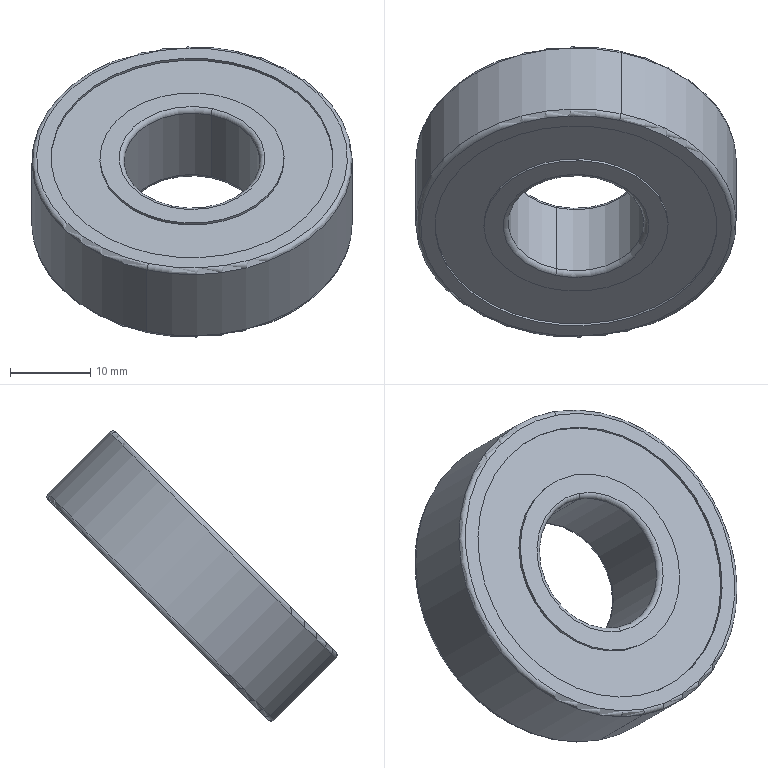Component | SolidWorks | AssemblyDriveAxis-1_6203-2 | 1 solid | 26 faces | box 40 x 36.27 x 36.27 mm | volume 11947 mm3 | cylinder 12 | torus 8 | plane 6 | commonest cylinder face diameters 35.2 x4 23 x4 40 x2 17 x2
build123d program:
from build123d import *


with BuildPart() as part:
    # Sketch1 → Revolve1 (revolve)
    with BuildSketch(Plane.XY, mode=Mode.PRIVATE) as revolve1_sk:
        with BuildLine():
            Line((0, 19.4), (0, 17.6))
            Line((0, 17.6), (0.342, 17.6))
            Line((0.342, 17.6), (0.342, 11.5))
            Line((0.342, 11.5), (0, 11.5))
            Line((0, 11.5), (0, 9.1))
            ThreePointArc((0, 9.1), (0.1757, 8.676), (0.6, 8.5))
            Line((0.6, 8.5), (11.4, 8.5))
            ThreePointArc((11.4, 8.5), (11.824, 8.676), (12, 9.1))
            Line((12, 9.1), (12, 11.5))
            Line((12, 11.5), (11.658, 11.5))
            Line((11.658, 11.5), (11.658, 17.6))
            Line((11.658, 17.6), (12, 17.6))
            Line((12, 17.6), (12, 19.4))
            ThreePointArc((12, 19.4), (11.824, 19.824), (11.4, 20))
            Line((11.4, 20), (0.6, 20))
            ThreePointArc((0.6, 20), (0.1757, 19.824), (0, 19.4))
        make_face()
    revolve(revolve1_sk.sketch.rotate(Axis((12, 0, 0), (-1, 0, 0)), 270), axis=Axis((12, 0, 0), (-1, 0, 0)))


solid = part.part

# Placed as in the assembly
solid = solid.moved(Location((-102, 782.057, 125.043), (135, 86.529, 90)))
STEP:
#1=COLOUR_RGB('',0.7922,0.8196,0.9333);
#2=FILL_AREA_STYLE_COLOUR('',#1);
#3=FILL_AREA_STYLE('',(#2));
#4=SURFACE_STYLE_FILL_AREA(#3);
#5=SURFACE_SIDE_STYLE('',(#4));
#6=SURFACE_STYLE_USAGE(.BOTH.,#5);
#7=PRESENTATION_STYLE_ASSIGNMENT((#6));
#8=CARTESIAN_POINT('',(-4.237,30.239,4.405));
#9=VERTEX_POINT('',#8);
#10=CARTESIAN_POINT('',(-3.794,31.307,5.474));
#11=VERTEX_POINT('',#10);
#12=CARTESIAN_POINT('',(-4.016,30.773,4.94));
#13=DIRECTION('',(-0.,-0.7071,0.7071));
#14=DIRECTION('',(-0.2811,-0.6786,-0.6786));
#15=AXIS2_PLACEMENT_3D('',#12,#13,#14);
#16=CIRCLE('',#15,0.7874);
#17=EDGE_CURVE('',#9,#11,#16,.T.);
#18=ORIENTED_EDGE('',*,*,#17,.T.);
#19=CARTESIAN_POINT('',(-3.794,31.007,5.775));
#20=VERTEX_POINT('',#19);
#21=CARTESIAN_POINT('',(-3.794,31.324,5.457));
#22=DIRECTION('',(-0.,-0.7071,0.7071));
#23=VECTOR('',#22,39.37);
#24=LINE('',#21,#23);
#25=EDGE_CURVE('',#11,#20,#24,.T.);
#26=ORIENTED_EDGE('',*,*,#25,.T.);
#27=CARTESIAN_POINT('',(-4.237,29.938,4.706));
#28=VERTEX_POINT('',#27);
#29=CARTESIAN_POINT('',(-4.016,30.472,5.24));
#30=DIRECTION('',(-0.,-0.7071,0.7071));
#31=DIRECTION('',(-0.2811,-0.6786,-0.6786));
#32=AXIS2_PLACEMENT_3D('',#29,#30,#31);
#33=CIRCLE('',#32,0.7874);
#34=EDGE_CURVE('',#28,#20,#33,.T.);
#35=ORIENTED_EDGE('',*,*,#34,.F.);
#36=CARTESIAN_POINT('',(-4.237,30.255,4.389));
#37=DIRECTION('',(-0.,-0.7071,0.7071));
#38=VECTOR('',#37,39.37);
#39=LINE('',#36,#38);
#40=EDGE_CURVE('',#9,#28,#39,.T.);
#41=ORIENTED_EDGE('',*,*,#40,.F.);
#42=EDGE_LOOP('',(#18,#26,#35,#41));
#43=FACE_OUTER_BOUND('',#42,.T.);
#44=CARTESIAN_POINT('',(-4.016,30.79,4.923));
#45=DIRECTION('',(-0.,-0.7071,0.7071));
#46=DIRECTION('',(-0.2811,-0.6786,-0.6786));
#47=AXIS2_PLACEMENT_3D('',#44,#45,#46);
#48=CYLINDRICAL_SURFACE('',#47,0.7874);
#49=ADVANCED_FACE('',(#43),#48,.T.);
#50=CARTESIAN_POINT('',(-4.23,30.271,4.405));
#51=VERTEX_POINT('',#50);
#52=CARTESIAN_POINT('',(-3.801,31.308,5.441));
#53=VERTEX_POINT('',#52);
#54=CARTESIAN_POINT('',(-4.016,30.79,4.923));
#55=DIRECTION('',(-0.,-0.7071,0.7071));
#56=DIRECTION('',(-0.2811,-0.6786,-0.6786));
#57=AXIS2_PLACEMENT_3D('',#54,#55,#56);
#58=CIRCLE('',#57,0.7638);
#59=EDGE_CURVE('',#51,#53,#58,.T.);
#60=ORIENTED_EDGE('',*,*,#59,.T.);
#61=CARTESIAN_POINT('',(-3.801,31.291,5.458));
#62=DIRECTION('',(0.9597,-0.1988,-0.1988));
#63=DIRECTION('',(-0.2028,0.,-0.9792));
#64=AXIS2_PLACEMENT_3D('',#61,#62,#63);
#65=CIRCLE('',#64,0.02362);
#66=EDGE_CURVE('',#53,#11,#65,.T.);
#67=ORIENTED_EDGE('',*,*,#66,.T.);
#68=ORIENTED_EDGE('',*,*,#17,.F.);
#69=CARTESIAN_POINT('',(-4.23,30.255,4.421));
#70=DIRECTION('',(-0.9597,0.1988,0.1988));
#71=DIRECTION('',(0.2028,0.,0.9792));
#72=AXIS2_PLACEMENT_3D('',#69,#70,#71);
#73=CIRCLE('',#72,0.02362);
#74=EDGE_CURVE('',#51,#9,#73,.T.);
#75=ORIENTED_EDGE('',*,*,#74,.F.);
#76=EDGE_LOOP('',(#60,#67,#68,#75));
#77=FACE_OUTER_BOUND('',#76,.T.);
#78=CARTESIAN_POINT('',(-4.016,30.773,4.94));
#79=DIRECTION('',(-0.,-0.7071,0.7071));
#80=DIRECTION('',(-0.2811,-0.6786,-0.6786));
#81=AXIS2_PLACEMENT_3D('',#78,#79,#80);
#82=TOROIDAL_SURFACE('',#81,0.7638,0.02362);
#83=ADVANCED_FACE('',(#77),#82,.T.);
#84=CARTESIAN_POINT('',(-3.821,31.26,5.393));
#85=VERTEX_POINT('',#84);
#86=CARTESIAN_POINT('',(-4.211,30.319,4.453));
#87=VERTEX_POINT('',#86);
#88=CARTESIAN_POINT('',(-4.016,30.79,4.923));
#89=DIRECTION('',(-0.,-0.7071,0.7071));
#90=DIRECTION('',(-0.2811,-0.6786,-0.6786));
#91=AXIS2_PLACEMENT_3D('',#88,#89,#90);
#92=CIRCLE('',#91,0.6929);
#93=EDGE_CURVE('',#85,#87,#92,.T.);
#94=ORIENTED_EDGE('',*,*,#93,.F.);
#95=CARTESIAN_POINT('',(-3.821,31.25,5.403));
#96=VERTEX_POINT('',#95);
#97=CARTESIAN_POINT('',(-3.821,31.26,5.393));
#98=DIRECTION('',(-0.,-0.7071,0.7071));
#99=VECTOR('',#98,39.37);
#100=LINE('',#97,#99);
#101=EDGE_CURVE('',#85,#96,#100,.T.);
#102=ORIENTED_EDGE('',*,*,#101,.T.);
#103=CARTESIAN_POINT('',(-4.211,30.31,4.462));
#104=VERTEX_POINT('',#103);
#105=CARTESIAN_POINT('',(-4.016,30.78,4.932));
#106=DIRECTION('',(-0.,-0.7071,0.7071));
#107=DIRECTION('',(-0.2811,-0.6786,-0.6786));
#108=AXIS2_PLACEMENT_3D('',#105,#106,#107);
#109=CIRCLE('',#108,0.6929);
#110=EDGE_CURVE('',#96,#104,#109,.T.);
#111=ORIENTED_EDGE('',*,*,#110,.T.);
#112=CARTESIAN_POINT('',(-4.211,30.319,4.453));
#113=DIRECTION('',(-0.,-0.7071,0.7071));
#114=VECTOR('',#113,39.37);
#115=LINE('',#112,#114);
#116=EDGE_CURVE('',#87,#104,#115,.T.);
#117=ORIENTED_EDGE('',*,*,#116,.F.);
#118=EDGE_LOOP('',(#94,#102,#111,#117));
#119=FACE_OUTER_BOUND('',#118,.T.);
#120=CARTESIAN_POINT('',(-4.016,30.79,4.923));
#121=DIRECTION('',(-0.,-0.7071,0.7071));
#122=DIRECTION('',(-0.2811,-0.6786,-0.6786));
#123=AXIS2_PLACEMENT_3D('',#120,#121,#122);
#124=CYLINDRICAL_SURFACE('',#123,0.6929);
#125=ADVANCED_FACE('',(#119),#124,.F.);
#126=CARTESIAN_POINT('',(-4.143,30.482,4.616));
#127=VERTEX_POINT('',#126);
#128=CARTESIAN_POINT('',(-3.888,31.097,5.23));
#129=VERTEX_POINT('',#128);
#130=CARTESIAN_POINT('',(-4.016,30.79,4.923));
#131=DIRECTION('',(-0.,-0.7071,0.7071));
#132=DIRECTION('',(-0.2811,-0.6786,-0.6786));
#133=AXIS2_PLACEMENT_3D('',#130,#131,#132);
#134=CIRCLE('',#133,0.4528);
#135=EDGE_CURVE('',#127,#129,#134,.T.);
#136=ORIENTED_EDGE('',*,*,#135,.T.);
#137=CARTESIAN_POINT('',(-3.888,31.087,5.24));
#138=VERTEX_POINT('',#137);
#139=CARTESIAN_POINT('',(-3.888,31.097,5.23));
#140=DIRECTION('',(-0.,-0.7071,0.7071));
#141=VECTOR('',#140,39.37);
#142=LINE('',#139,#141);
#143=EDGE_CURVE('',#129,#138,#142,.T.);
#144=ORIENTED_EDGE('',*,*,#143,.T.);
#145=CARTESIAN_POINT('',(-4.143,30.473,4.625));
#146=VERTEX_POINT('',#145);
#147=CARTESIAN_POINT('',(-4.016,30.78,4.932));
#148=DIRECTION('',(-0.,-0.7071,0.7071));
#149=DIRECTION('',(-0.2811,-0.6786,-0.6786));
#150=AXIS2_PLACEMENT_3D('',#147,#148,#149);
#151=CIRCLE('',#150,0.4528);
#152=EDGE_CURVE('',#146,#138,#151,.T.);
#153=ORIENTED_EDGE('',*,*,#152,.F.);
#154=CARTESIAN_POINT('',(-4.143,30.482,4.616));
#155=DIRECTION('',(-0.,-0.7071,0.7071));
#156=VECTOR('',#155,39.37);
#157=LINE('',#154,#156);
#158=EDGE_CURVE('',#127,#146,#157,.T.);
#159=ORIENTED_EDGE('',*,*,#158,.F.);
#160=EDGE_LOOP('',(#136,#144,#153,#159));
#161=FACE_OUTER_BOUND('',#160,.T.);
#162=CARTESIAN_POINT('',(-4.016,30.79,4.923));
#163=DIRECTION('',(-0.,-0.7071,0.7071));
#164=DIRECTION('',(-0.2811,-0.6786,-0.6786));
#165=AXIS2_PLACEMENT_3D('',#162,#163,#164);
#166=CYLINDRICAL_SURFACE('',#165,0.4528);
#167=ADVANCED_FACE('',(#161),#166,.T.);
#168=CARTESIAN_POINT('',(-4.11,30.546,4.713));
#169=VERTEX_POINT('',#168);
#170=CARTESIAN_POINT('',(-3.922,31.,5.167));
#171=VERTEX_POINT('',#170);
#172=CARTESIAN_POINT('',(-4.016,30.773,4.94));
#173=DIRECTION('',(-0.,-0.7071,0.7071));
#174=DIRECTION('',(-0.2811,-0.6786,-0.6786));
#175=AXIS2_PLACEMENT_3D('',#172,#173,#174);
#176=CIRCLE('',#175,0.3346);
#177=EDGE_CURVE('',#169,#171,#176,.T.);
#178=ORIENTED_EDGE('',*,*,#177,.T.);
#179=CARTESIAN_POINT('',(-3.915,31.033,5.166));
#180=VERTEX_POINT('',#179);
#181=CARTESIAN_POINT('',(-3.915,31.016,5.183));
#182=DIRECTION('',(0.9597,-0.1988,-0.1988));
#183=DIRECTION('',(-0.2028,0.,-0.9792));
#184=AXIS2_PLACEMENT_3D('',#181,#182,#183);
#185=CIRCLE('',#184,0.02362);
#186=EDGE_CURVE('',#171,#180,#185,.T.);
#187=ORIENTED_EDGE('',*,*,#186,.T.);
#188=CARTESIAN_POINT('',(-4.116,30.547,4.68));
#189=VERTEX_POINT('',#188);
#190=CARTESIAN_POINT('',(-4.016,30.79,4.923));
#191=DIRECTION('',(-0.,-0.7071,0.7071));
#192=DIRECTION('',(-0.2811,-0.6786,-0.6786));
#193=AXIS2_PLACEMENT_3D('',#190,#191,#192);
#194=CIRCLE('',#193,0.3583);
#195=EDGE_CURVE('',#189,#180,#194,.T.);
#196=ORIENTED_EDGE('',*,*,#195,.F.);
#197=CARTESIAN_POINT('',(-4.116,30.53,4.697));
#198=DIRECTION('',(-0.9597,0.1988,0.1988));
#199=DIRECTION('',(0.2028,0.,0.9792));
#200=AXIS2_PLACEMENT_3D('',#197,#198,#199);
#201=CIRCLE('',#200,0.02362);
#202=EDGE_CURVE('',#169,#189,#201,.T.);
#203=ORIENTED_EDGE('',*,*,#202,.F.);
#204=EDGE_LOOP('',(#178,#187,#196,#203));
#205=FACE_OUTER_BOUND('',#204,.T.);
#206=CARTESIAN_POINT('',(-4.016,30.773,4.94));
#207=DIRECTION('',(-0.,-0.7071,0.7071));
#208=DIRECTION('',(-0.2811,-0.6786,-0.6786));
#209=AXIS2_PLACEMENT_3D('',#206,#207,#208);
#210=TOROIDAL_SURFACE('',#209,0.3583,0.02362);
#211=ADVANCED_FACE('',(#205),#210,.T.);
#212=CARTESIAN_POINT('',(-4.016,30.773,4.94));
#213=DIRECTION('',(-0.,-0.7071,0.7071));
#214=DIRECTION('',(-0.2811,-0.6786,-0.6786));
#215=AXIS2_PLACEMENT_3D('',#212,#213,#214);
#216=CIRCLE('',#215,0.3346);
#217=EDGE_CURVE('',#171,#169,#216,.T.);
#218=ORIENTED_EDGE('',*,*,#217,.F.);
#219=CARTESIAN_POINT('',(-3.922,30.699,5.467));
#220=VERTEX_POINT('',#219);
#221=CARTESIAN_POINT('',(-3.922,31.017,5.15));
#222=DIRECTION('',(-0.,-0.7071,0.7071));
#223=VECTOR('',#222,39.37);
#224=LINE('',#221,#223);
#225=EDGE_CURVE('',#171,#220,#224,.T.);
#226=ORIENTED_EDGE('',*,*,#225,.T.);
#227=CARTESIAN_POINT('',(-4.11,30.245,5.013));
#228=VERTEX_POINT('',#227);
#229=CARTESIAN_POINT('',(-4.016,30.472,5.24));
#230=DIRECTION('',(-0.,-0.7071,0.7071));
#231=DIRECTION('',(-0.2811,-0.6786,-0.6786));
#232=AXIS2_PLACEMENT_3D('',#229,#230,#231);
#233=CIRCLE('',#232,0.3346);
#234=EDGE_CURVE('',#220,#228,#233,.T.);
#235=ORIENTED_EDGE('',*,*,#234,.T.);
#236=CARTESIAN_POINT('',(-4.11,30.563,4.696));
#237=DIRECTION('',(-0.,-0.7071,0.7071));
#238=VECTOR('',#237,39.37);
#239=LINE('',#236,#238);
#240=EDGE_CURVE('',#169,#228,#239,.T.);
#241=ORIENTED_EDGE('',*,*,#240,.F.);
#242=EDGE_LOOP('',(#218,#226,#235,#241));
#243=FACE_OUTER_BOUND('',#242,.T.);
#244=CARTESIAN_POINT('',(-4.016,30.79,4.923));
#245=DIRECTION('',(-0.,-0.7071,0.7071));
#246=DIRECTION('',(-0.2811,-0.6786,-0.6786));
#247=AXIS2_PLACEMENT_3D('',#244,#245,#246);
#248=CYLINDRICAL_SURFACE('',#247,0.3346);
#249=ADVANCED_FACE('',(#243),#248,.F.);
#250=CARTESIAN_POINT('',(-4.116,30.212,5.014));
#251=VERTEX_POINT('',#250);
#252=CARTESIAN_POINT('',(-3.915,30.699,5.5));
#253=VERTEX_POINT('',#252);
#254=CARTESIAN_POINT('',(-4.016,30.456,5.257));
#255=DIRECTION('',(-0.,-0.7071,0.7071));
#256=DIRECTION('',(-0.2811,-0.6786,-0.6786));
#257=AXIS2_PLACEMENT_3D('',#254,#255,#256);
#258=CIRCLE('',#257,0.3583);
#259=EDGE_CURVE('',#251,#253,#258,.T.);
#260=ORIENTED_EDGE('',*,*,#259,.T.);
#261=CARTESIAN_POINT('',(-3.915,30.715,5.483));
#262=DIRECTION('',(0.9597,-0.1988,-0.1988));
#263=DIRECTION('',(-0.2028,0.,-0.9792));
#264=AXIS2_PLACEMENT_3D('',#261,#262,#263);
#265=CIRCLE('',#264,0.02362);
#266=EDGE_CURVE('',#253,#220,#265,.T.);
#267=ORIENTED_EDGE('',*,*,#266,.T.);
#268=CARTESIAN_POINT('',(-4.016,30.472,5.24));
#269=DIRECTION('',(-0.,-0.7071,0.7071));
#270=DIRECTION('',(-0.2811,-0.6786,-0.6786));
#271=AXIS2_PLACEMENT_3D('',#268,#269,#270);
#272=CIRCLE('',#271,0.3346);
#273=EDGE_CURVE('',#228,#220,#272,.T.);
#274=ORIENTED_EDGE('',*,*,#273,.F.);
#275=CARTESIAN_POINT('',(-4.116,30.229,4.997));
#276=DIRECTION('',(-0.9597,0.1988,0.1988));
#277=DIRECTION('',(0.2028,0.,0.9792));
#278=AXIS2_PLACEMENT_3D('',#275,#276,#277);
#279=CIRCLE('',#278,0.02362);
#280=EDGE_CURVE('',#251,#228,#279,.T.);
#281=ORIENTED_EDGE('',*,*,#280,.F.);
#282=EDGE_LOOP('',(#260,#267,#274,#281));
#283=FACE_OUTER_BOUND('',#282,.T.);
#284=CARTESIAN_POINT('',(-4.016,30.472,5.24));
#285=DIRECTION('',(-0.,-0.7071,0.7071));
#286=DIRECTION('',(-0.2811,-0.6786,-0.6786));
#287=AXIS2_PLACEMENT_3D('',#284,#285,#286);
#288=TOROIDAL_SURFACE('',#287,0.3583,0.02362);
#289=ADVANCED_FACE('',(#283),#288,.T.);
#290=CARTESIAN_POINT('',(-4.143,30.158,4.94));
#291=VERTEX_POINT('',#290);
#292=CARTESIAN_POINT('',(-3.888,30.772,5.555));
#293=VERTEX_POINT('',#292);
#294=CARTESIAN_POINT('',(-4.016,30.465,5.247));
#295=DIRECTION('',(-0.,-0.7071,0.7071));
#296=DIRECTION('',(-0.2811,-0.6786,-0.6786));
#297=AXIS2_PLACEMENT_3D('',#294,#295,#296);
#298=CIRCLE('',#297,0.4528);
#299=EDGE_CURVE('',#291,#293,#298,.T.);
#300=ORIENTED_EDGE('',*,*,#299,.T.);
#301=CARTESIAN_POINT('',(-3.888,30.763,5.564));
#302=VERTEX_POINT('',#301);
#303=CARTESIAN_POINT('',(-3.888,31.097,5.23));
#304=DIRECTION('',(-0.,-0.7071,0.7071));
#305=VECTOR('',#304,39.37);
#306=LINE('',#303,#305);
#307=EDGE_CURVE('',#293,#302,#306,.T.);
#308=ORIENTED_EDGE('',*,*,#307,.T.);
#309=CARTESIAN_POINT('',(-4.143,30.148,4.95));
#310=VERTEX_POINT('',#309);
#311=CARTESIAN_POINT('',(-4.016,30.456,5.257));
#312=DIRECTION('',(-0.,-0.7071,0.7071));
#313=DIRECTION('',(-0.2811,-0.6786,-0.6786));
#314=AXIS2_PLACEMENT_3D('',#311,#312,#313);
#315=CIRCLE('',#314,0.4528);
#316=EDGE_CURVE('',#310,#302,#315,.T.);
#317=ORIENTED_EDGE('',*,*,#316,.F.);
#318=CARTESIAN_POINT('',(-4.143,30.482,4.616));
#319=DIRECTION('',(-0.,-0.7071,0.7071));
#320=VECTOR('',#319,39.37);
#321=LINE('',#318,#320);
#322=EDGE_CURVE('',#291,#310,#321,.T.);
#323=ORIENTED_EDGE('',*,*,#322,.F.);
#324=EDGE_LOOP('',(#300,#308,#317,#323));
#325=FACE_OUTER_BOUND('',#324,.T.);
#326=CARTESIAN_POINT('',(-4.016,30.79,4.923));
#327=DIRECTION('',(-0.,-0.7071,0.7071));
#328=DIRECTION('',(-0.2811,-0.6786,-0.6786));
#329=AXIS2_PLACEMENT_3D('',#326,#327,#328);
#330=CYLINDRICAL_SURFACE('',#329,0.4528);
#331=ADVANCED_FACE('',(#325),#330,.T.);
#332=CARTESIAN_POINT('',(-3.821,30.935,5.718));
#333=VERTEX_POINT('',#332);
#334=CARTESIAN_POINT('',(-4.211,29.995,4.777));
#335=VERTEX_POINT('',#334);
#336=CARTESIAN_POINT('',(-4.016,30.465,5.247));
#337=DIRECTION('',(-0.,-0.7071,0.7071));
#338=DIRECTION('',(-0.2811,-0.6786,-0.6786));
#339=AXIS2_PLACEMENT_3D('',#336,#337,#338);
#340=CIRCLE('',#339,0.6929);
#341=EDGE_CURVE('',#333,#335,#340,.T.);
#342=ORIENTED_EDGE('',*,*,#341,.F.);
#343=CARTESIAN_POINT('',(-3.821,30.926,5.727));
#344=VERTEX_POINT('',#343);
#345=CARTESIAN_POINT('',(-3.821,31.26,5.393));
#346=DIRECTION('',(-0.,-0.7071,0.7071));
#347=VECTOR('',#346,39.37);
#348=LINE('',#345,#347);
#349=EDGE_CURVE('',#333,#344,#348,.T.);
#350=ORIENTED_EDGE('',*,*,#349,.T.);
#351=CARTESIAN_POINT('',(-4.211,29.985,4.787));
#352=VERTEX_POINT('',#351);
#353=CARTESIAN_POINT('',(-4.016,30.456,5.257));
#354=DIRECTION('',(-0.,-0.7071,0.7071));
#355=DIRECTION('',(-0.2811,-0.6786,-0.6786));
#356=AXIS2_PLACEMENT_3D('',#353,#354,#355);
#357=CIRCLE('',#356,0.6929);
#358=EDGE_CURVE('',#344,#352,#357,.T.);
#359=ORIENTED_EDGE('',*,*,#358,.T.);
#360=CARTESIAN_POINT('',(-4.211,30.319,4.453));
#361=DIRECTION('',(-0.,-0.7071,0.7071));
#362=VECTOR('',#361,39.37);
#363=LINE('',#360,#362);
#364=EDGE_CURVE('',#335,#352,#363,.T.);
#365=ORIENTED_EDGE('',*,*,#364,.F.);
#366=EDGE_LOOP('',(#342,#350,#359,#365));
#367=FACE_OUTER_BOUND('',#366,.T.);
#368=CARTESIAN_POINT('',(-4.016,30.79,4.923));
#369=DIRECTION('',(-0.,-0.7071,0.7071));
#370=DIRECTION('',(-0.2811,-0.6786,-0.6786));
#371=AXIS2_PLACEMENT_3D('',#368,#369,#370);
#372=CYLINDRICAL_SURFACE('',#371,0.6929);
#373=ADVANCED_FACE('',(#367),#372,.F.);
#374=ORIENTED_EDGE('',*,*,#34,.T.);
#375=CARTESIAN_POINT('',(-3.801,30.974,5.775));
#376=VERTEX_POINT('',#375);
#377=CARTESIAN_POINT('',(-3.801,30.991,5.759));
#378=DIRECTION('',(0.9597,-0.1988,-0.1988));
#379=DIRECTION('',(-0.2028,0.,-0.9792));
#380=AXIS2_PLACEMENT_3D('',#377,#378,#379);
#381=CIRCLE('',#380,0.02362);
#382=EDGE_CURVE('',#20,#376,#381,.T.);
#383=ORIENTED_EDGE('',*,*,#382,.T.);
#384=CARTESIAN_POINT('',(-4.23,29.937,4.739));
#385=VERTEX_POINT('',#384);
#386=CARTESIAN_POINT('',(-4.016,30.456,5.257));
#387=DIRECTION('',(-0.,-0.7071,0.7071));
#388=DIRECTION('',(-0.2811,-0.6786,-0.6786));
#389=AXIS2_PLACEMENT_3D('',#386,#387,#388);
#390=CIRCLE('',#389,0.7638);
#391=EDGE_CURVE('',#385,#376,#390,.T.);
#392=ORIENTED_EDGE('',*,*,#391,.F.);
#393=CARTESIAN_POINT('',(-4.23,29.954,4.722));
#394=DIRECTION('',(-0.9597,0.1988,0.1988));
#395=DIRECTION('',(0.2028,0.,0.9792));
#396=AXIS2_PLACEMENT_3D('',#393,#394,#395);
#397=CIRCLE('',#396,0.02362);
#398=EDGE_CURVE('',#28,#385,#397,.T.);
#399=ORIENTED_EDGE('',*,*,#398,.F.);
#400=EDGE_LOOP('',(#374,#383,#392,#399));
#401=FACE_OUTER_BOUND('',#400,.T.);
#402=CARTESIAN_POINT('',(-4.016,30.472,5.24));
#403=DIRECTION('',(-0.,-0.7071,0.7071));
#404=DIRECTION('',(-0.2811,-0.6786,-0.6786));
#405=AXIS2_PLACEMENT_3D('',#402,#403,#404);
#406=TOROIDAL_SURFACE('',#405,0.7638,0.02362);
#407=ADVANCED_FACE('',(#401),#406,.T.);
#408=ORIENTED_EDGE('',*,*,#382,.F.);
#409=CARTESIAN_POINT('',(-4.016,30.472,5.24));
#410=DIRECTION('',(-0.,-0.7071,0.7071));
#411=DIRECTION('',(-0.2811,-0.6786,-0.6786));
#412=AXIS2_PLACEMENT_3D('',#409,#410,#411);
#413=CIRCLE('',#412,0.7874);
#414=EDGE_CURVE('',#20,#28,#413,.T.);
#415=ORIENTED_EDGE('',*,*,#414,.T.);
#416=ORIENTED_EDGE('',*,*,#398,.T.);
#417=CARTESIAN_POINT('',(-4.016,30.456,5.257));
#418=DIRECTION('',(-0.,-0.7071,0.7071));
#419=DIRECTION('',(-0.2811,-0.6786,-0.6786));
#420=AXIS2_PLACEMENT_3D('',#417,#418,#419);
#421=CIRCLE('',#420,0.7638);
#422=EDGE_CURVE('',#376,#385,#421,.T.);
#423=ORIENTED_EDGE('',*,*,#422,.F.);
#424=EDGE_LOOP('',(#408,#415,#416,#423));
#425=FACE_OUTER_BOUND('',#424,.T.);
#426=CARTESIAN_POINT('',(-4.016,30.472,5.24));
#427=DIRECTION('',(-0.,-0.7071,0.7071));
#428=DIRECTION('',(-0.2811,-0.6786,-0.6786));
#429=AXIS2_PLACEMENT_3D('',#426,#427,#428);
#430=TOROIDAL_SURFACE('',#429,0.7638,0.02362);
#431=ADVANCED_FACE('',(#425),#430,.T.);
#432=CARTESIAN_POINT('',(-4.016,30.456,5.257));
#433=DIRECTION('',(-0.,-0.7071,0.7071));
#434=DIRECTION('',(-0.2811,-0.6786,-0.6786));
#435=AXIS2_PLACEMENT_3D('',#432,#433,#434);
#436=CIRCLE('',#435,0.6929);
#437=EDGE_CURVE('',#352,#344,#436,.T.);
#438=ORIENTED_EDGE('',*,*,#437,.F.);
#439=ORIENTED_EDGE('',*,*,#358,.F.);
#440=EDGE_LOOP('',(#438,#439));
#441=FACE_BOUND('',#440,.T.);
#442=ORIENTED_EDGE('',*,*,#391,.T.);
#443=ORIENTED_EDGE('',*,*,#422,.T.);
#444=EDGE_LOOP('',(#442,#443));
#445=FACE_OUTER_BOUND('',#444,.T.);
#446=CARTESIAN_POINT('',(-3.283,30.304,5.105));
#447=DIRECTION('',(0.,0.7071,-0.7071));
#448=DIRECTION('',(0.2811,0.6786,0.6786));
#449=AXIS2_PLACEMENT_3D('',#446,#447,#448);
#450=PLANE('',#449);
#451=ADVANCED_FACE('',(#441,#445),#450,.F.);
#452=ORIENTED_EDGE('',*,*,#349,.F.);
#453=CARTESIAN_POINT('',(-4.016,30.465,5.247));
#454=DIRECTION('',(-0.,-0.7071,0.7071));
#455=DIRECTION('',(-0.2811,-0.6786,-0.6786));
#456=AXIS2_PLACEMENT_3D('',#453,#454,#455);
#457=CIRCLE('',#456,0.6929);
#458=EDGE_CURVE('',#335,#333,#457,.T.);
#459=ORIENTED_EDGE('',*,*,#458,.F.);
#460=ORIENTED_EDGE('',*,*,#364,.T.);
#461=ORIENTED_EDGE('',*,*,#437,.T.);
#462=EDGE_LOOP('',(#452,#459,#460,#461));
#463=FACE_OUTER_BOUND('',#462,.T.);
#464=CARTESIAN_POINT('',(-4.016,30.79,4.923));
#465=DIRECTION('',(-0.,-0.7071,0.7071));
#466=DIRECTION('',(-0.2811,-0.6786,-0.6786));
#467=AXIS2_PLACEMENT_3D('',#464,#465,#466);
#468=CYLINDRICAL_SURFACE('',#467,0.6929);
#469=ADVANCED_FACE('',(#463),#468,.F.);
#470=ORIENTED_EDGE('',*,*,#299,.F.);
#471=CARTESIAN_POINT('',(-4.016,30.465,5.247));
#472=DIRECTION('',(-0.,-0.7071,0.7071));
#473=DIRECTION('',(-0.2811,-0.6786,-0.6786));
#474=AXIS2_PLACEMENT_3D('',#471,#472,#473);
#475=CIRCLE('',#474,0.4528);
#476=EDGE_CURVE('',#293,#291,#475,.T.);
#477=ORIENTED_EDGE('',*,*,#476,.F.);
#478=EDGE_LOOP('',(#470,#477));
#479=FACE_BOUND('',#478,.T.);
#480=ORIENTED_EDGE('',*,*,#458,.T.);
#481=ORIENTED_EDGE('',*,*,#341,.T.);
#482=EDGE_LOOP('',(#480,#481));
#483=FACE_OUTER_BOUND('',#482,.T.);
#484=CARTESIAN_POINT('',(-3.351,30.327,5.11));
#485=DIRECTION('',(0.,0.7071,-0.7071));
#486=DIRECTION('',(0.2811,0.6786,0.6786));
#487=AXIS2_PLACEMENT_3D('',#484,#485,#486);
#488=PLANE('',#487);
#489=ADVANCED_FACE('',(#479,#483),#488,.F.);
#490=ORIENTED_EDGE('',*,*,#307,.F.);
#491=ORIENTED_EDGE('',*,*,#476,.T.);
#492=ORIENTED_EDGE('',*,*,#322,.T.);
#493=CARTESIAN_POINT('',(-4.016,30.456,5.257));
#494=DIRECTION('',(-0.,-0.7071,0.7071));
#495=DIRECTION('',(-0.2811,-0.6786,-0.6786));
#496=AXIS2_PLACEMENT_3D('',#493,#494,#495);
#497=CIRCLE('',#496,0.4528);
#498=EDGE_CURVE('',#302,#310,#497,.T.);
#499=ORIENTED_EDGE('',*,*,#498,.F.);
#500=EDGE_LOOP('',(#490,#491,#492,#499));
#501=FACE_OUTER_BOUND('',#500,.T.);
#502=CARTESIAN_POINT('',(-4.016,30.79,4.923));
#503=DIRECTION('',(-0.,-0.7071,0.7071));
#504=DIRECTION('',(-0.2811,-0.6786,-0.6786));
#505=AXIS2_PLACEMENT_3D('',#502,#503,#504);
#506=CYLINDRICAL_SURFACE('',#505,0.4528);
#507=ADVANCED_FACE('',(#501),#506,.T.);
#508=ORIENTED_EDGE('',*,*,#259,.F.);
#509=CARTESIAN_POINT('',(-4.016,30.456,5.257));
#510=DIRECTION('',(-0.,-0.7071,0.7071));
#511=DIRECTION('',(-0.2811,-0.6786,-0.6786));
#512=AXIS2_PLACEMENT_3D('',#509,#510,#511);
#513=CIRCLE('',#512,0.3583);
#514=EDGE_CURVE('',#253,#251,#513,.T.);
#515=ORIENTED_EDGE('',*,*,#514,.F.);
#516=EDGE_LOOP('',(#508,#515));
#517=FACE_BOUND('',#516,.T.);
#518=ORIENTED_EDGE('',*,*,#316,.T.);
#519=ORIENTED_EDGE('',*,*,#498,.T.);
#520=EDGE_LOOP('',(#518,#519));
#521=FACE_OUTER_BOUND('',#520,.T.);
#522=CARTESIAN_POINT('',(-3.581,30.366,5.167));
#523=DIRECTION('',(0.,0.7071,-0.7071));
#524=DIRECTION('',(0.2811,0.6786,0.6786));
#525=AXIS2_PLACEMENT_3D('',#522,#523,#524);
#526=PLANE('',#525);
#527=ADVANCED_FACE('',(#517,#521),#526,.F.);
#528=ORIENTED_EDGE('',*,*,#266,.F.);
#529=ORIENTED_EDGE('',*,*,#514,.T.);
#530=ORIENTED_EDGE('',*,*,#280,.T.);
#531=ORIENTED_EDGE('',*,*,#234,.F.);
#532=EDGE_LOOP('',(#528,#529,#530,#531));
#533=FACE_OUTER_BOUND('',#532,.T.);
#534=CARTESIAN_POINT('',(-4.016,30.472,5.24));
#535=DIRECTION('',(-0.,-0.7071,0.7071));
#536=DIRECTION('',(-0.2811,-0.6786,-0.6786));
#537=AXIS2_PLACEMENT_3D('',#534,#535,#536);
#538=TOROIDAL_SURFACE('',#537,0.3583,0.02362);
#539=ADVANCED_FACE('',(#533),#538,.T.);
#540=ORIENTED_EDGE('',*,*,#225,.F.);
#541=ORIENTED_EDGE('',*,*,#177,.F.);
#542=ORIENTED_EDGE('',*,*,#240,.T.);
#543=ORIENTED_EDGE('',*,*,#273,.T.);
#544=EDGE_LOOP('',(#540,#541,#542,#543));
#545=FACE_OUTER_BOUND('',#544,.T.);
#546=CARTESIAN_POINT('',(-4.016,30.79,4.923));
#547=DIRECTION('',(-0.,-0.7071,0.7071));
#548=DIRECTION('',(-0.2811,-0.6786,-0.6786));
#549=AXIS2_PLACEMENT_3D('',#546,#547,#548);
#550=CYLINDRICAL_SURFACE('',#549,0.3346);
#551=ADVANCED_FACE('',(#545),#550,.F.);
#552=ORIENTED_EDGE('',*,*,#186,.F.);
#553=ORIENTED_EDGE('',*,*,#217,.T.);
#554=ORIENTED_EDGE('',*,*,#202,.T.);
#555=CARTESIAN_POINT('',(-4.016,30.79,4.923));
#556=DIRECTION('',(-0.,-0.7071,0.7071));
#557=DIRECTION('',(-0.2811,-0.6786,-0.6786));
#558=AXIS2_PLACEMENT_3D('',#555,#556,#557);
#559=CIRCLE('',#558,0.3583);
#560=EDGE_CURVE('',#180,#189,#559,.T.);
#561=ORIENTED_EDGE('',*,*,#560,.F.);
#562=EDGE_LOOP('',(#552,#553,#554,#561));
#563=FACE_OUTER_BOUND('',#562,.T.);
#564=CARTESIAN_POINT('',(-4.016,30.773,4.94));
#565=DIRECTION('',(-0.,-0.7071,0.7071));
#566=DIRECTION('',(-0.2811,-0.6786,-0.6786));
#567=AXIS2_PLACEMENT_3D('',#564,#565,#566);
#568=TOROIDAL_SURFACE('',#567,0.3583,0.02362);
#569=ADVANCED_FACE('',(#563),#568,.T.);
#570=ORIENTED_EDGE('',*,*,#135,.F.);
#571=CARTESIAN_POINT('',(-4.016,30.79,4.923));
#572=DIRECTION('',(-0.,-0.7071,0.7071));
#573=DIRECTION('',(-0.2811,-0.6786,-0.6786));
#574=AXIS2_PLACEMENT_3D('',#571,#572,#573);
#575=CIRCLE('',#574,0.4528);
#576=EDGE_CURVE('',#129,#127,#575,.T.);
#577=ORIENTED_EDGE('',*,*,#576,.F.);
#578=EDGE_LOOP('',(#570,#577));
#579=FACE_OUTER_BOUND('',#578,.T.);
#580=ORIENTED_EDGE('',*,*,#195,.T.);
#581=ORIENTED_EDGE('',*,*,#560,.T.);
#582=EDGE_LOOP('',(#580,#581));
#583=FACE_BOUND('',#582,.T.);
#584=CARTESIAN_POINT('',(-3.672,30.718,4.852));
#585=DIRECTION('',(-0.,-0.7071,0.7071));
#586=DIRECTION('',(-0.2811,-0.6786,-0.6786));
#587=AXIS2_PLACEMENT_3D('',#584,#585,#586);
#588=PLANE('',#587);
#589=ADVANCED_FACE('',(#579,#583),#588,.F.);
#590=ORIENTED_EDGE('',*,*,#143,.F.);
#591=ORIENTED_EDGE('',*,*,#576,.T.);
#592=ORIENTED_EDGE('',*,*,#158,.T.);
#593=CARTESIAN_POINT('',(-4.016,30.78,4.932));
#594=DIRECTION('',(-0.,-0.7071,0.7071));
#595=DIRECTION('',(-0.2811,-0.6786,-0.6786));
#596=AXIS2_PLACEMENT_3D('',#593,#594,#595);
#597=CIRCLE('',#596,0.4528);
#598=EDGE_CURVE('',#138,#146,#597,.T.);
#599=ORIENTED_EDGE('',*,*,#598,.F.);
#600=EDGE_LOOP('',(#590,#591,#592,#599));
#601=FACE_OUTER_BOUND('',#600,.T.);
#602=CARTESIAN_POINT('',(-4.016,30.79,4.923));
#603=DIRECTION('',(-0.,-0.7071,0.7071));
#604=DIRECTION('',(-0.2811,-0.6786,-0.6786));
#605=AXIS2_PLACEMENT_3D('',#602,#603,#604);
#606=CYLINDRICAL_SURFACE('',#605,0.4528);
#607=ADVANCED_FACE('',(#601),#606,.T.);
#608=CARTESIAN_POINT('',(-4.016,30.78,4.932));
#609=DIRECTION('',(-0.,-0.7071,0.7071));
#610=DIRECTION('',(-0.2811,-0.6786,-0.6786));
#611=AXIS2_PLACEMENT_3D('',#608,#609,#610);
#612=CIRCLE('',#611,0.6929);
#613=EDGE_CURVE('',#104,#96,#612,.T.);
#614=ORIENTED_EDGE('',*,*,#613,.F.);
#615=ORIENTED_EDGE('',*,*,#110,.F.);
#616=EDGE_LOOP('',(#614,#615));
#617=FACE_OUTER_BOUND('',#616,.T.);
#618=ORIENTED_EDGE('',*,*,#152,.T.);
#619=ORIENTED_EDGE('',*,*,#598,.T.);
#620=EDGE_LOOP('',(#618,#619));
#621=FACE_BOUND('',#620,.T.);
#622=CARTESIAN_POINT('',(-3.581,30.69,4.842));
#623=DIRECTION('',(-0.,-0.7071,0.7071));
#624=DIRECTION('',(-0.2811,-0.6786,-0.6786));
#625=AXIS2_PLACEMENT_3D('',#622,#623,#624);
#626=PLANE('',#625);
#627=ADVANCED_FACE('',(#617,#621),#626,.F.);
#628=ORIENTED_EDGE('',*,*,#101,.F.);
#629=CARTESIAN_POINT('',(-4.016,30.79,4.923));
#630=DIRECTION('',(-0.,-0.7071,0.7071));
#631=DIRECTION('',(-0.2811,-0.6786,-0.6786));
#632=AXIS2_PLACEMENT_3D('',#629,#630,#631);
#633=CIRCLE('',#632,0.6929);
#634=EDGE_CURVE('',#87,#85,#633,.T.);
#635=ORIENTED_EDGE('',*,*,#634,.F.);
#636=ORIENTED_EDGE('',*,*,#116,.T.);
#637=ORIENTED_EDGE('',*,*,#613,.T.);
#638=EDGE_LOOP('',(#628,#635,#636,#637));
#639=FACE_OUTER_BOUND('',#638,.T.);
#640=CARTESIAN_POINT('',(-4.016,30.79,4.923));
#641=DIRECTION('',(-0.,-0.7071,0.7071));
#642=DIRECTION('',(-0.2811,-0.6786,-0.6786));
#643=AXIS2_PLACEMENT_3D('',#640,#641,#642);
#644=CYLINDRICAL_SURFACE('',#643,0.6929);
#645=ADVANCED_FACE('',(#639),#644,.F.);
#646=ORIENTED_EDGE('',*,*,#59,.F.);
#647=CARTESIAN_POINT('',(-4.016,30.79,4.923));
#648=DIRECTION('',(-0.,-0.7071,0.7071));
#649=DIRECTION('',(-0.2811,-0.6786,-0.6786));
#650=AXIS2_PLACEMENT_3D('',#647,#648,#649);
#651=CIRCLE('',#650,0.7638);
#652=EDGE_CURVE('',#53,#51,#651,.T.);
#653=ORIENTED_EDGE('',*,*,#652,.F.);
#654=EDGE_LOOP('',(#646,#653));
#655=FACE_OUTER_BOUND('',#654,.T.);
#656=ORIENTED_EDGE('',*,*,#634,.T.);
#657=ORIENTED_EDGE('',*,*,#93,.T.);
#658=EDGE_LOOP('',(#656,#657));
#659=FACE_BOUND('',#658,.T.);
#660=CARTESIAN_POINT('',(-3.351,30.652,4.785));
#661=DIRECTION('',(-0.,-0.7071,0.7071));
#662=DIRECTION('',(-0.2811,-0.6786,-0.6786));
#663=AXIS2_PLACEMENT_3D('',#660,#661,#662);
#664=PLANE('',#663);
#665=ADVANCED_FACE('',(#655,#659),#664,.F.);
#666=ORIENTED_EDGE('',*,*,#66,.F.);
#667=ORIENTED_EDGE('',*,*,#652,.T.);
#668=ORIENTED_EDGE('',*,*,#74,.T.);
#669=CARTESIAN_POINT('',(-4.016,30.773,4.94));
#670=DIRECTION('',(-0.,-0.7071,0.7071));
#671=DIRECTION('',(-0.2811,-0.6786,-0.6786));
#672=AXIS2_PLACEMENT_3D('',#669,#670,#671);
#673=CIRCLE('',#672,0.7874);
#674=EDGE_CURVE('',#11,#9,#673,.T.);
#675=ORIENTED_EDGE('',*,*,#674,.F.);
#676=EDGE_LOOP('',(#666,#667,#668,#675));
#677=FACE_OUTER_BOUND('',#676,.T.);
#678=CARTESIAN_POINT('',(-4.016,30.773,4.94));
#679=DIRECTION('',(-0.,-0.7071,0.7071));
#680=DIRECTION('',(-0.2811,-0.6786,-0.6786));
#681=AXIS2_PLACEMENT_3D('',#678,#679,#680);
#682=TOROIDAL_SURFACE('',#681,0.7638,0.02362);
#683=ADVANCED_FACE('',(#677),#682,.T.);
#684=ORIENTED_EDGE('',*,*,#25,.F.);
#685=ORIENTED_EDGE('',*,*,#674,.T.);
#686=ORIENTED_EDGE('',*,*,#40,.T.);
#687=ORIENTED_EDGE('',*,*,#414,.F.);
#688=EDGE_LOOP('',(#684,#685,#686,#687));
#689=FACE_OUTER_BOUND('',#688,.T.);
#690=CARTESIAN_POINT('',(-4.016,30.79,4.923));
#691=DIRECTION('',(-0.,-0.7071,0.7071));
#692=DIRECTION('',(-0.2811,-0.6786,-0.6786));
#693=AXIS2_PLACEMENT_3D('',#690,#691,#692);
#694=CYLINDRICAL_SURFACE('',#693,0.7874);
#695=ADVANCED_FACE('',(#689),#694,.T.);
#696=CLOSED_SHELL('',(#49,#83,#125,#167,#211,#249,#289,#331,#373,#407,#431,#451,#469,#489,#507,#527,#539,#551,#569,#589,#607,#627,#645,#665,#683,#695));
#697=MANIFOLD_SOLID_BREP('',#696);
#698=STYLED_ITEM('',(#7),#697);
#699=PRESENTATION_LAYER_ASSIGNMENT('','',(#698));
#700=CARTESIAN_POINT('',(0.,0.,0.));
#701=DIRECTION('',(0.,0.,1.));
#702=DIRECTION('',(1.,0.,0.));
#703=AXIS2_PLACEMENT_3D('',#700,#701,#702);
#704=(LENGTH_UNIT()NAMED_UNIT(*)SI_UNIT($,.METRE.));
#705=LENGTH_MEASURE_WITH_UNIT(LENGTH_MEASURE(0.0254),#704);
#706=DIMENSIONAL_EXPONENTS(1.,0.,0.,0.,0.,0.,0.);
#707=(CONVERSION_BASED_UNIT('',#705)LENGTH_UNIT()NAMED_UNIT(#706));
#708=UNCERTAINTY_MEASURE_WITH_UNIT(LENGTH_MEASURE(0.00001),#707,'','');
#709=(NAMED_UNIT(*)PLANE_ANGLE_UNIT()SI_UNIT($,.RADIAN.));
#710=(NAMED_UNIT(*)SI_UNIT($,.STERADIAN.)SOLID_ANGLE_UNIT());
#711=(GEOMETRIC_REPRESENTATION_CONTEXT(3)GLOBAL_UNCERTAINTY_ASSIGNED_CONTEXT((#708))GLOBAL_UNIT_ASSIGNED_CONTEXT((#707,#709,#710))REPRESENTATION_CONTEXT('',''));
#712=ADVANCED_BREP_SHAPE_REPRESENTATION('',(#697,#703),#711);
#713=(LENGTH_UNIT()NAMED_UNIT(*)SI_UNIT($,.METRE.));
#714=LENGTH_MEASURE_WITH_UNIT(LENGTH_MEASURE(0.0254),#713);
#715=DIMENSIONAL_EXPONENTS(1.,0.,0.,0.,0.,0.,0.);
#716=(CONVERSION_BASED_UNIT('',#714)LENGTH_UNIT()NAMED_UNIT(#715));
#717=UNCERTAINTY_MEASURE_WITH_UNIT(LENGTH_MEASURE(0.00001),#716,'','');
#718=(NAMED_UNIT(*)PLANE_ANGLE_UNIT()SI_UNIT($,.RADIAN.));
#719=(NAMED_UNIT(*)SI_UNIT($,.STERADIAN.)SOLID_ANGLE_UNIT());
#720=(GEOMETRIC_REPRESENTATION_CONTEXT(3)GLOBAL_UNCERTAINTY_ASSIGNED_CONTEXT((#717))GLOBAL_UNIT_ASSIGNED_CONTEXT((#716,#718,#719))REPRESENTATION_CONTEXT('',''));
#721=MECHANICAL_DESIGN_GEOMETRIC_PRESENTATION_REPRESENTATION('',(#698),#720);